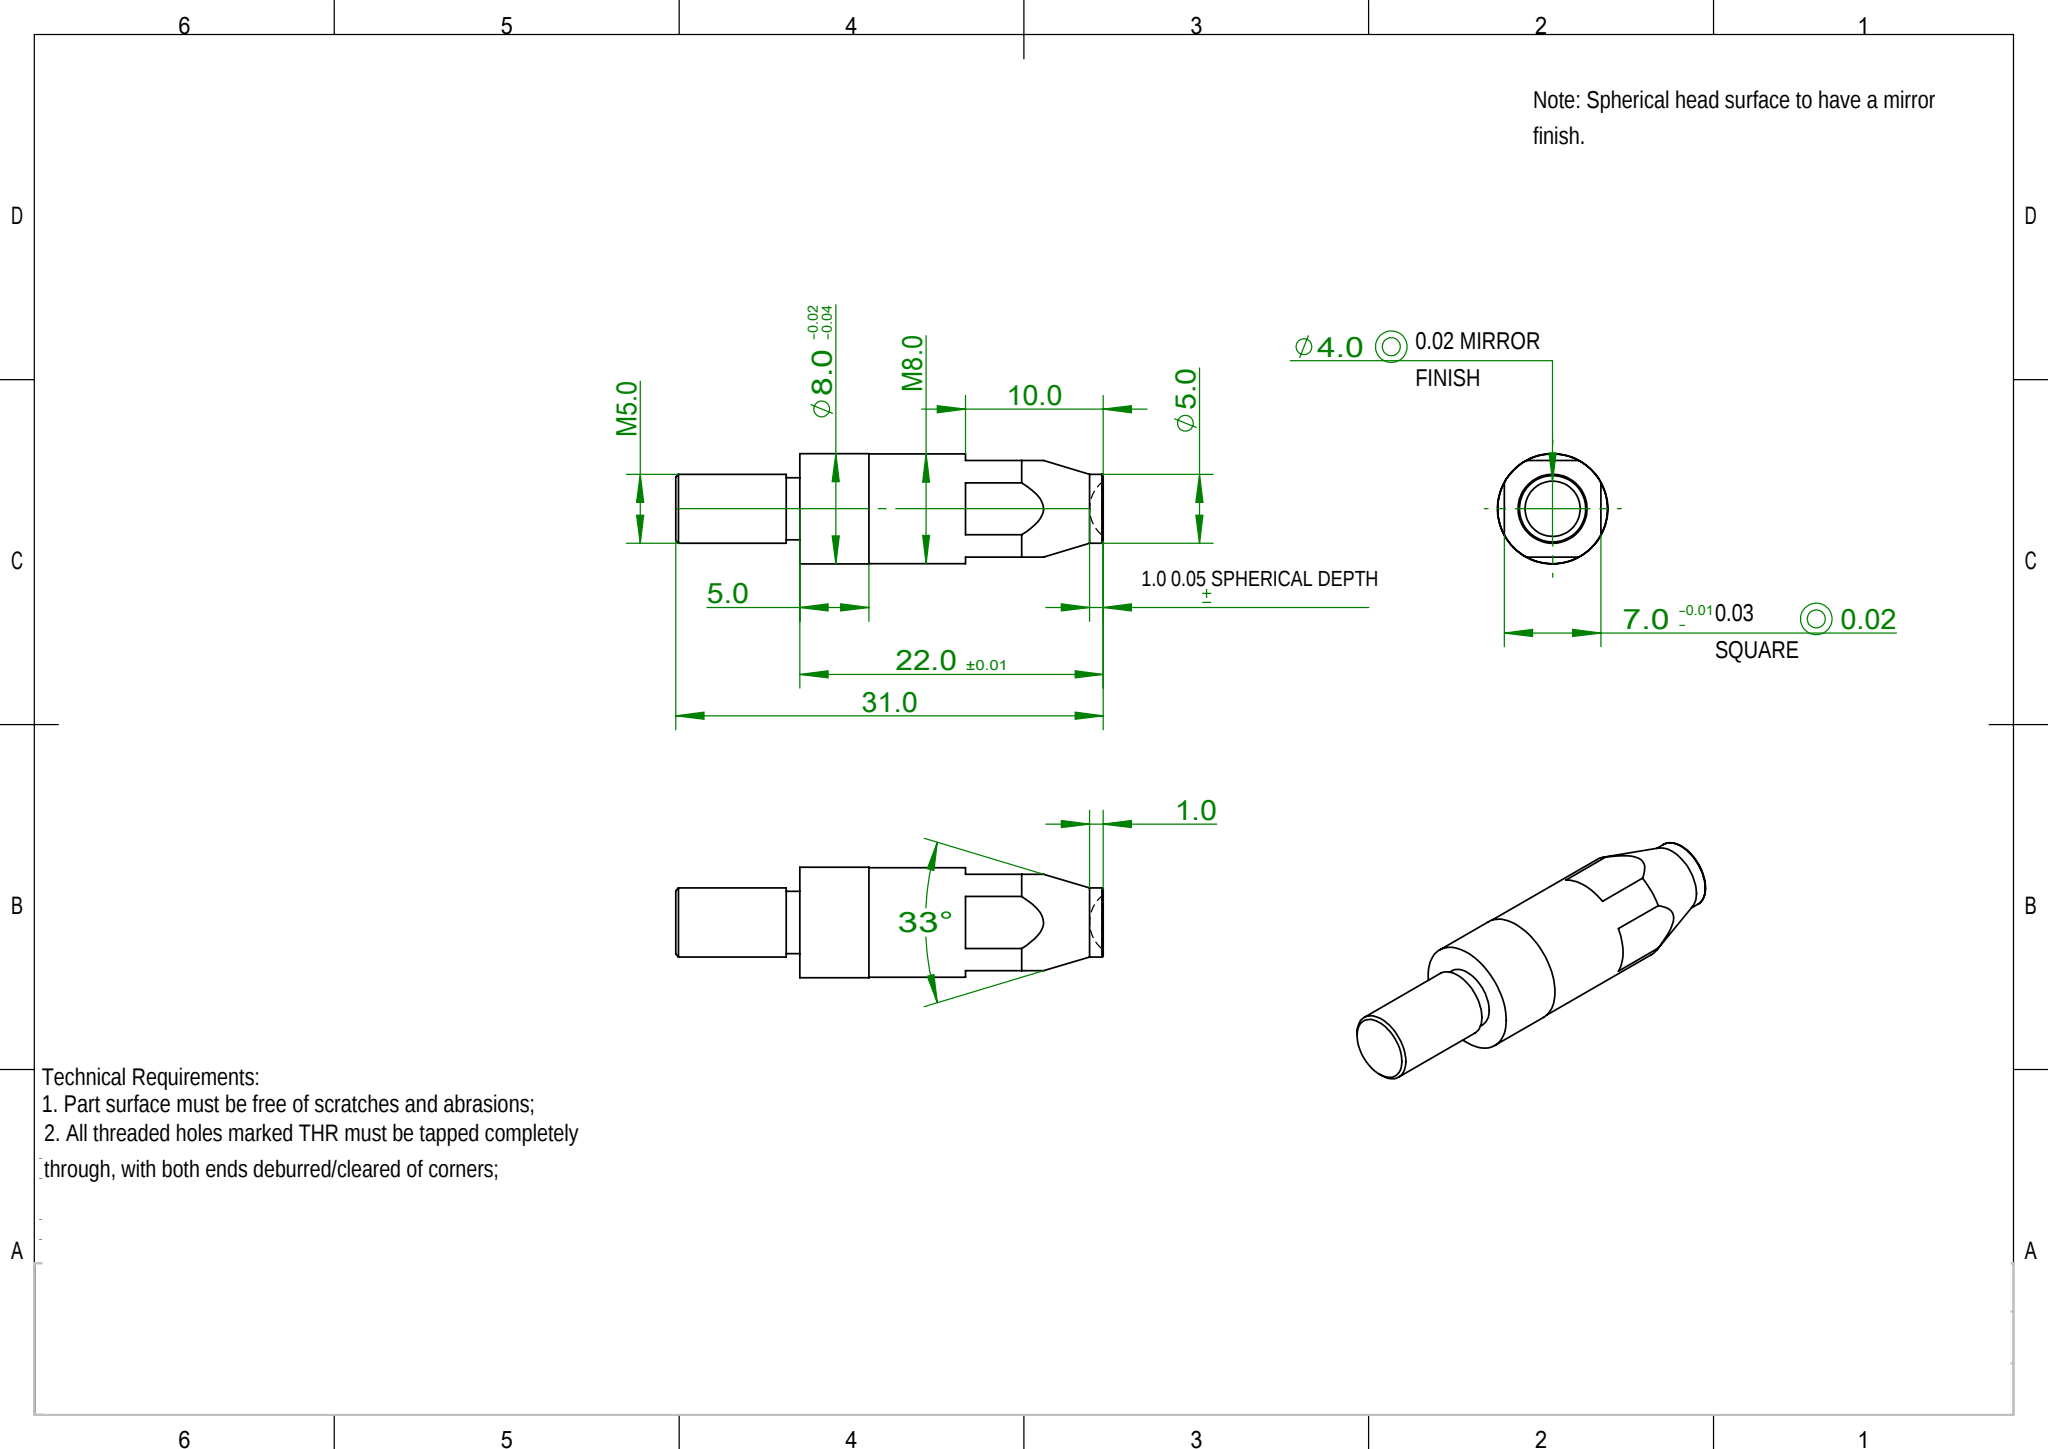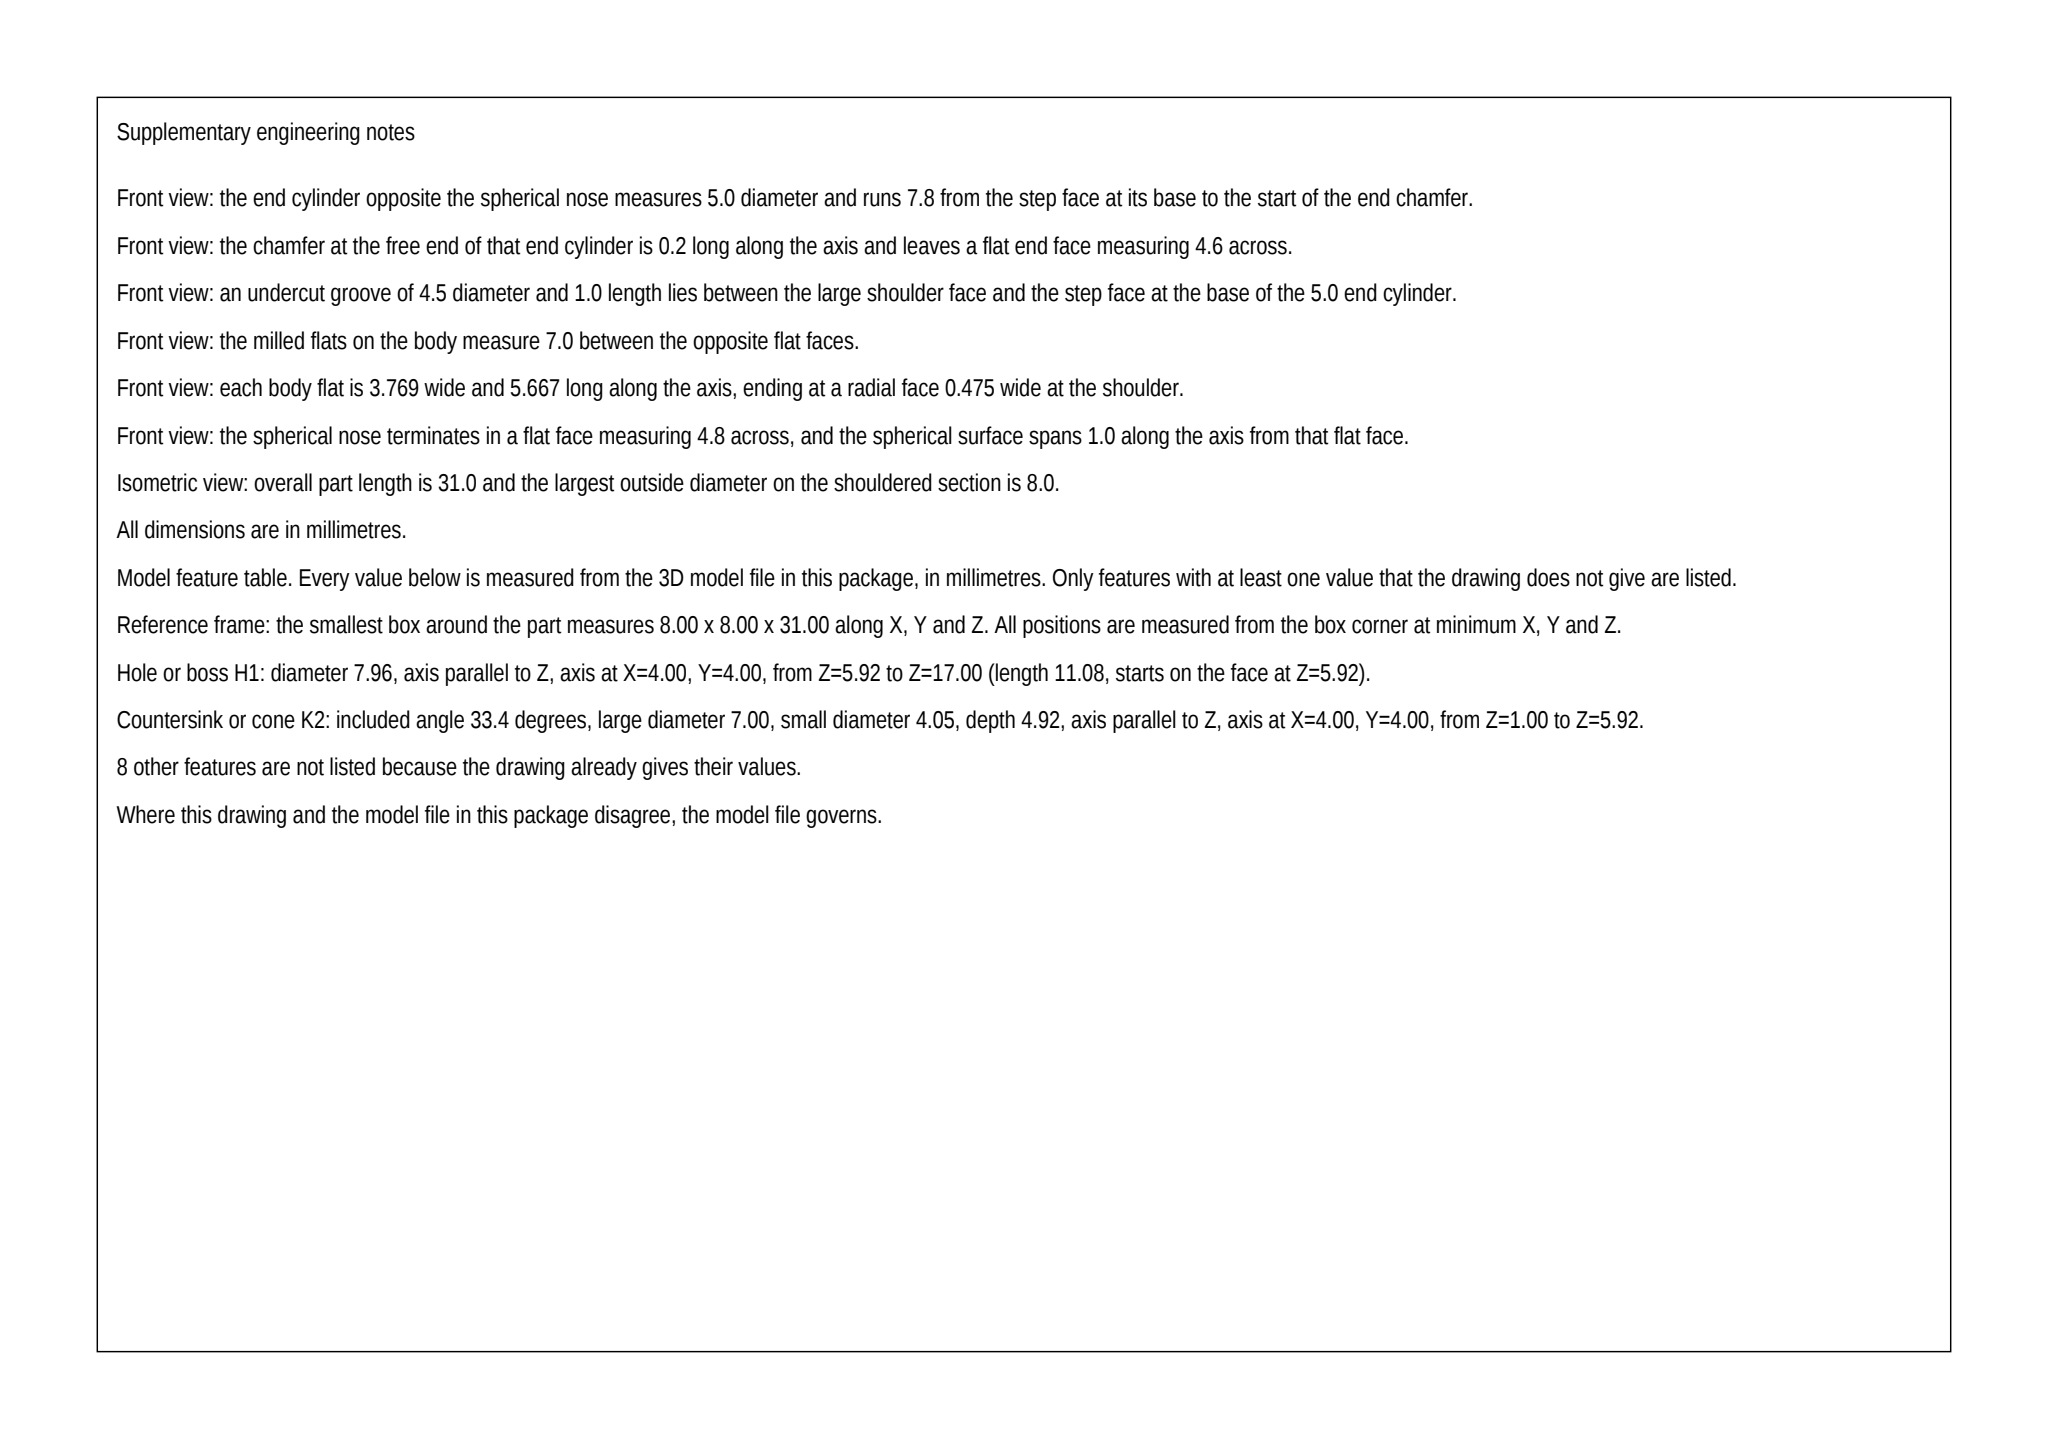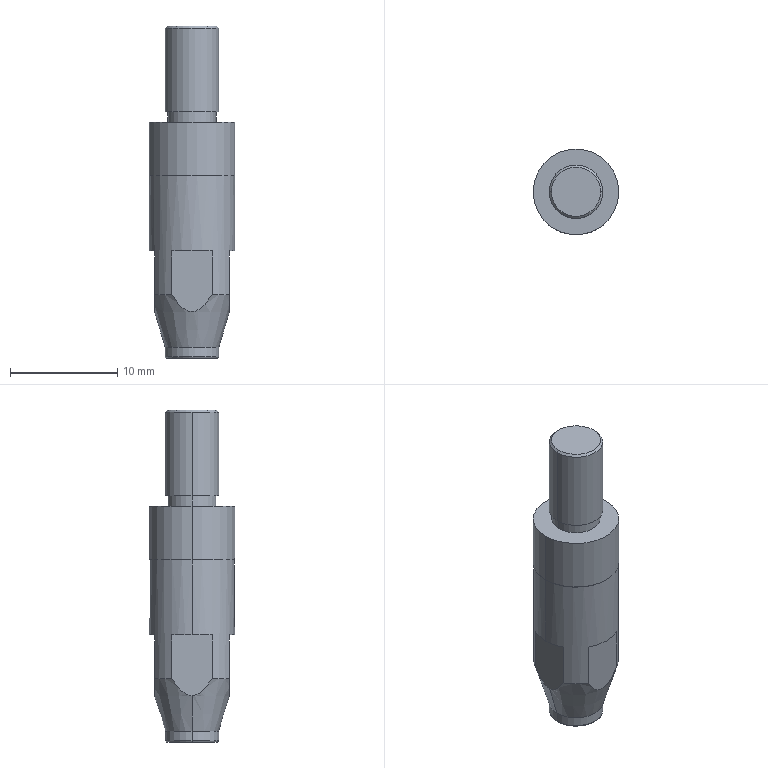Part | SolidWorks | mm | 1 solid | 31 faces | box 8 x 8 x 31 mm | volume 1129 mm3 | plane 13 | cylinder 10 | cone 4 | torus 2 | sphere 2 | commonest cylinder face diameters 5 x4 4.5 x2 8 x2 7.95 x2